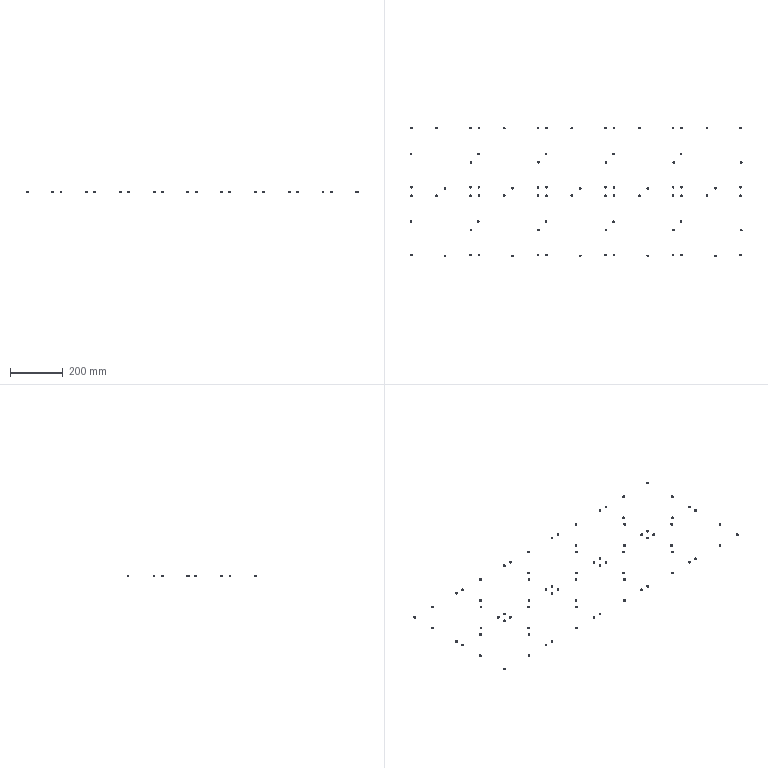Component | SolidWorks | P16BoxWeldment-1_M3RivetNut-1 | 80 solids | 480 faces | box 1258 x 490 x 3.5 mm | volume 5938 mm3 | cylinder 320 | plane 160 | commonest cylinder face diameters 3 x160 6 x160
build123d program:
from build123d import *

# Parameters (mm, degrees)
SKETCH1_R           = 3
SKETCH1_R_2         = 1.5
BOSS_EXTRUDE1_DEPTH = 3.5


with BuildPart() as part:
    # Sketch1 → Boss-Extrude1 (new body)
    # profile 1 of 80: a face of its own
    with BuildSketch(Plane.XY):
        with Locations((-352, 0)):
            Circle(SKETCH1_R)
        with Locations((-352, 0)):
            Circle(SKETCH1_R_2, mode=Mode.SUBTRACT)
    # profile 2 of 80: a face of its own
    with BuildSketch(Plane.XY):
        with Locations((-256, 0)):
            Circle(SKETCH1_R)
        with Locations((-256, 0)):
            Circle(SKETCH1_R_2, mode=Mode.SUBTRACT)
    # profile 3 of 80: a face of its own
    with BuildSketch(Plane.XY):
        with Locations((-128, 0)):
            Circle(SKETCH1_R)
        with Locations((-128, 0)):
            Circle(SKETCH1_R_2, mode=Mode.SUBTRACT)
    # profile 4 of 80: a face of its own
    with BuildSketch(Plane.XY):
        with Locations((-354, -98)):
            Circle(SKETCH1_R)
        with Locations((-354, -98)):
            Circle(SKETCH1_R_2, mode=Mode.SUBTRACT)
    # profile 5 of 80: a face of its own
    with BuildSketch(Plane.XY):
        with Locations((-126, -130)):
            Circle(SKETCH1_R)
        with Locations((-126, -130)):
            Circle(SKETCH1_R_2, mode=Mode.SUBTRACT)
    # profile 6 of 80: a face of its own
    with BuildSketch(Plane.XY):
        with Locations((-128, -224)):
            Circle(SKETCH1_R)
        with Locations((-128, -224)):
            Circle(SKETCH1_R_2, mode=Mode.SUBTRACT)
    # profile 7 of 80: a face of its own
    with BuildSketch(Plane.XY):
        with Locations((-224, -228)):
            Circle(SKETCH1_R)
        with Locations((-224, -228)):
            Circle(SKETCH1_R_2, mode=Mode.SUBTRACT)
    # profile 8 of 80: a face of its own
    with BuildSketch(Plane.XY):
        with Locations((-352, -224)):
            Circle(SKETCH1_R)
        with Locations((-352, -224)):
            Circle(SKETCH1_R_2, mode=Mode.SUBTRACT)
    # profile 9 of 80: a face of its own
    with BuildSketch(Plane.XY):
        with Locations((-96, 0)):
            Circle(SKETCH1_R)
        with Locations((-96, 0)):
            Circle(SKETCH1_R_2, mode=Mode.SUBTRACT)
    # profile 10 of 80: a face of its own
    with BuildSketch(Plane.XY):
        Circle(SKETCH1_R)
        Circle(SKETCH1_R_2, mode=Mode.SUBTRACT)
    # profile 11 of 80: a face of its own
    with BuildSketch(Plane.XY):
        with Locations((128, 0)):
            Circle(SKETCH1_R)
        with Locations((128, 0)):
            Circle(SKETCH1_R_2, mode=Mode.SUBTRACT)
    # profile 12 of 80: a face of its own
    with BuildSketch(Plane.XY):
        with Locations((-98, -98)):
            Circle(SKETCH1_R)
        with Locations((-98, -98)):
            Circle(SKETCH1_R_2, mode=Mode.SUBTRACT)
    # profile 13 of 80: a face of its own
    with BuildSketch(Plane.XY):
        with Locations((130, -130)):
            Circle(SKETCH1_R)
        with Locations((130, -130)):
            Circle(SKETCH1_R_2, mode=Mode.SUBTRACT)
    # profile 14 of 80: a face of its own
    with BuildSketch(Plane.XY):
        with Locations((128, -224)):
            Circle(SKETCH1_R)
        with Locations((128, -224)):
            Circle(SKETCH1_R_2, mode=Mode.SUBTRACT)
    # profile 15 of 80: a face of its own
    with BuildSketch(Plane.XY):
        with Locations((32, -228)):
            Circle(SKETCH1_R)
        with Locations((32, -228)):
            Circle(SKETCH1_R_2, mode=Mode.SUBTRACT)
    # profile 16 of 80: a face of its own
    with BuildSketch(Plane.XY):
        with Locations((-96, -224)):
            Circle(SKETCH1_R)
        with Locations((-96, -224)):
            Circle(SKETCH1_R_2, mode=Mode.SUBTRACT)
    # profile 17 of 80: a face of its own
    with BuildSketch(Plane.XY):
        with Locations((160, 0)):
            Circle(SKETCH1_R)
        with Locations((160, 0)):
            Circle(SKETCH1_R_2, mode=Mode.SUBTRACT)
    # profile 18 of 80: a face of its own
    with BuildSketch(Plane.XY):
        with Locations((256, 0)):
            Circle(SKETCH1_R)
        with Locations((256, 0)):
            Circle(SKETCH1_R_2, mode=Mode.SUBTRACT)
    # profile 19 of 80: a face of its own
    with BuildSketch(Plane.XY):
        with Locations((384, 0)):
            Circle(SKETCH1_R)
        with Locations((384, 0)):
            Circle(SKETCH1_R_2, mode=Mode.SUBTRACT)
    # profile 20 of 80: a face of its own
    with BuildSketch(Plane.XY):
        with Locations((158, -98)):
            Circle(SKETCH1_R)
        with Locations((158, -98)):
            Circle(SKETCH1_R_2, mode=Mode.SUBTRACT)
    # profile 21 of 80: a face of its own
    with BuildSketch(Plane.XY):
        with Locations((386, -130)):
            Circle(SKETCH1_R)
        with Locations((386, -130)):
            Circle(SKETCH1_R_2, mode=Mode.SUBTRACT)
    # profile 22 of 80: a face of its own
    with BuildSketch(Plane.XY):
        with Locations((384, -224)):
            Circle(SKETCH1_R)
        with Locations((384, -224)):
            Circle(SKETCH1_R_2, mode=Mode.SUBTRACT)
    # profile 23 of 80: a face of its own
    with BuildSketch(Plane.XY):
        with Locations((288, -228)):
            Circle(SKETCH1_R)
        with Locations((288, -228)):
            Circle(SKETCH1_R_2, mode=Mode.SUBTRACT)
    # profile 24 of 80: a face of its own
    with BuildSketch(Plane.XY):
        with Locations((160, -224)):
            Circle(SKETCH1_R)
        with Locations((160, -224)):
            Circle(SKETCH1_R_2, mode=Mode.SUBTRACT)
    # profile 25 of 80: a face of its own
    with BuildSketch(Plane.XY):
        with Locations((416, 0)):
            Circle(SKETCH1_R)
        with Locations((416, 0)):
            Circle(SKETCH1_R_2, mode=Mode.SUBTRACT)
    # profile 26 of 80: a face of its own
    with BuildSketch(Plane.XY):
        with Locations((512, 0)):
            Circle(SKETCH1_R)
        with Locations((512, 0)):
            Circle(SKETCH1_R_2, mode=Mode.SUBTRACT)
    # profile 27 of 80: a face of its own
    with BuildSketch(Plane.XY):
        with Locations((640, 0)):
            Circle(SKETCH1_R)
        with Locations((640, 0)):
            Circle(SKETCH1_R_2, mode=Mode.SUBTRACT)
    # profile 28 of 80: a face of its own
    with BuildSketch(Plane.XY):
        with Locations((414, -98)):
            Circle(SKETCH1_R)
        with Locations((414, -98)):
            Circle(SKETCH1_R_2, mode=Mode.SUBTRACT)
    # profile 29 of 80: a face of its own
    with BuildSketch(Plane.XY):
        with Locations((642, -130)):
            Circle(SKETCH1_R)
        with Locations((642, -130)):
            Circle(SKETCH1_R_2, mode=Mode.SUBTRACT)
    # profile 30 of 80: a face of its own
    with BuildSketch(Plane.XY):
        with Locations((640, -224)):
            Circle(SKETCH1_R)
        with Locations((640, -224)):
            Circle(SKETCH1_R_2, mode=Mode.SUBTRACT)
    # profile 31 of 80: a face of its own
    with BuildSketch(Plane.XY):
        with Locations((544, -228)):
            Circle(SKETCH1_R)
        with Locations((544, -228)):
            Circle(SKETCH1_R_2, mode=Mode.SUBTRACT)
    # profile 32 of 80: a face of its own
    with BuildSketch(Plane.XY):
        with Locations((416, -224)):
            Circle(SKETCH1_R)
        with Locations((416, -224)):
            Circle(SKETCH1_R_2, mode=Mode.SUBTRACT)
    # profile 33 of 80: a face of its own
    with BuildSketch(Plane.XY):
        with Locations((672, 0)):
            Circle(SKETCH1_R)
        with Locations((672, 0)):
            Circle(SKETCH1_R_2, mode=Mode.SUBTRACT)
    # profile 34 of 80: a face of its own
    with BuildSketch(Plane.XY):
        with Locations((768, 0)):
            Circle(SKETCH1_R)
        with Locations((768, 0)):
            Circle(SKETCH1_R_2, mode=Mode.SUBTRACT)
    # profile 35 of 80: a face of its own
    with BuildSketch(Plane.XY):
        with Locations((896, 0)):
            Circle(SKETCH1_R)
        with Locations((896, 0)):
            Circle(SKETCH1_R_2, mode=Mode.SUBTRACT)
    # profile 36 of 80: a face of its own
    with BuildSketch(Plane.XY):
        with Locations((670, -98)):
            Circle(SKETCH1_R)
        with Locations((670, -98)):
            Circle(SKETCH1_R_2, mode=Mode.SUBTRACT)
    # profile 37 of 80: a face of its own
    with BuildSketch(Plane.XY):
        with Locations((898, -130)):
            Circle(SKETCH1_R)
        with Locations((898, -130)):
            Circle(SKETCH1_R_2, mode=Mode.SUBTRACT)
    # profile 38 of 80: a face of its own
    with BuildSketch(Plane.XY):
        with Locations((896, -224)):
            Circle(SKETCH1_R)
        with Locations((896, -224)):
            Circle(SKETCH1_R_2, mode=Mode.SUBTRACT)
    # profile 39 of 80: a face of its own
    with BuildSketch(Plane.XY):
        with Locations((800, -228)):
            Circle(SKETCH1_R)
        with Locations((800, -228)):
            Circle(SKETCH1_R_2, mode=Mode.SUBTRACT)
    # profile 40 of 80: a face of its own
    with BuildSketch(Plane.XY):
        with Locations((672, -224)):
            Circle(SKETCH1_R)
        with Locations((672, -224)):
            Circle(SKETCH1_R_2, mode=Mode.SUBTRACT)
    # profile 41 of 80: a face of its own
    with BuildSketch(Plane.XY):
        with Locations((-352, -256)):
            Circle(SKETCH1_R)
        with Locations((-352, -256)):
            Circle(SKETCH1_R_2, mode=Mode.SUBTRACT)
    # profile 42 of 80: a face of its own
    with BuildSketch(Plane.XY):
        with Locations((-256, -256)):
            Circle(SKETCH1_R)
        with Locations((-256, -256)):
            Circle(SKETCH1_R_2, mode=Mode.SUBTRACT)
    # profile 43 of 80: a face of its own
    with BuildSketch(Plane.XY):
        with Locations((-128, -256)):
            Circle(SKETCH1_R)
        with Locations((-128, -256)):
            Circle(SKETCH1_R_2, mode=Mode.SUBTRACT)
    # profile 44 of 80: a face of its own
    with BuildSketch(Plane.XY):
        with Locations((-354, -354)):
            Circle(SKETCH1_R)
        with Locations((-354, -354)):
            Circle(SKETCH1_R_2, mode=Mode.SUBTRACT)
    # profile 45 of 80: a face of its own
    with BuildSketch(Plane.XY):
        with Locations((-126, -386)):
            Circle(SKETCH1_R)
        with Locations((-126, -386)):
            Circle(SKETCH1_R_2, mode=Mode.SUBTRACT)
    # profile 46 of 80: a face of its own
    with BuildSketch(Plane.XY):
        with Locations((-128, -480)):
            Circle(SKETCH1_R)
        with Locations((-128, -480)):
            Circle(SKETCH1_R_2, mode=Mode.SUBTRACT)
    # profile 47 of 80: a face of its own
    with BuildSketch(Plane.XY):
        with Locations((-224, -484)):
            Circle(SKETCH1_R)
        with Locations((-224, -484)):
            Circle(SKETCH1_R_2, mode=Mode.SUBTRACT)
    # profile 48 of 80: a face of its own
    with BuildSketch(Plane.XY):
        with Locations((-352, -480)):
            Circle(SKETCH1_R)
        with Locations((-352, -480)):
            Circle(SKETCH1_R_2, mode=Mode.SUBTRACT)
    # profile 49 of 80: a face of its own
    with BuildSketch(Plane.XY):
        with Locations((-96, -256)):
            Circle(SKETCH1_R)
        with Locations((-96, -256)):
            Circle(SKETCH1_R_2, mode=Mode.SUBTRACT)
    # profile 50 of 80: a face of its own
    with BuildSketch(Plane.XY):
        with Locations((0, -256)):
            Circle(SKETCH1_R)
        with Locations((0, -256)):
            Circle(SKETCH1_R_2, mode=Mode.SUBTRACT)
    # profile 51 of 80: a face of its own
    with BuildSketch(Plane.XY):
        with Locations((128, -256)):
            Circle(SKETCH1_R)
        with Locations((128, -256)):
            Circle(SKETCH1_R_2, mode=Mode.SUBTRACT)
    # profile 52 of 80: a face of its own
    with BuildSketch(Plane.XY):
        with Locations((-98, -354)):
            Circle(SKETCH1_R)
        with Locations((-98, -354)):
            Circle(SKETCH1_R_2, mode=Mode.SUBTRACT)
    # profile 53 of 80: a face of its own
    with BuildSketch(Plane.XY):
        with Locations((130, -386)):
            Circle(SKETCH1_R)
        with Locations((130, -386)):
            Circle(SKETCH1_R_2, mode=Mode.SUBTRACT)
    # profile 54 of 80: a face of its own
    with BuildSketch(Plane.XY):
        with Locations((128, -480)):
            Circle(SKETCH1_R)
        with Locations((128, -480)):
            Circle(SKETCH1_R_2, mode=Mode.SUBTRACT)
    # profile 55 of 80: a face of its own
    with BuildSketch(Plane.XY):
        with Locations((32, -484)):
            Circle(SKETCH1_R)
        with Locations((32, -484)):
            Circle(SKETCH1_R_2, mode=Mode.SUBTRACT)
    # profile 56 of 80: a face of its own
    with BuildSketch(Plane.XY):
        with Locations((-96, -480)):
            Circle(SKETCH1_R)
        with Locations((-96, -480)):
            Circle(SKETCH1_R_2, mode=Mode.SUBTRACT)
    # profile 57 of 80: a face of its own
    with BuildSketch(Plane.XY):
        with Locations((160, -256)):
            Circle(SKETCH1_R)
        with Locations((160, -256)):
            Circle(SKETCH1_R_2, mode=Mode.SUBTRACT)
    # profile 58 of 80: a face of its own
    with BuildSketch(Plane.XY):
        with Locations((256, -256)):
            Circle(SKETCH1_R)
        with Locations((256, -256)):
            Circle(SKETCH1_R_2, mode=Mode.SUBTRACT)
    # profile 59 of 80: a face of its own
    with BuildSketch(Plane.XY):
        with Locations((384, -256)):
            Circle(SKETCH1_R)
        with Locations((384, -256)):
            Circle(SKETCH1_R_2, mode=Mode.SUBTRACT)
    # profile 60 of 80: a face of its own
    with BuildSketch(Plane.XY):
        with Locations((158, -354)):
            Circle(SKETCH1_R)
        with Locations((158, -354)):
            Circle(SKETCH1_R_2, mode=Mode.SUBTRACT)
    # profile 61 of 80: a face of its own
    with BuildSketch(Plane.XY):
        with Locations((386, -386)):
            Circle(SKETCH1_R)
        with Locations((386, -386)):
            Circle(SKETCH1_R_2, mode=Mode.SUBTRACT)
    # profile 62 of 80: a face of its own
    with BuildSketch(Plane.XY):
        with Locations((384, -480)):
            Circle(SKETCH1_R)
        with Locations((384, -480)):
            Circle(SKETCH1_R_2, mode=Mode.SUBTRACT)
    # profile 63 of 80: a face of its own
    with BuildSketch(Plane.XY):
        with Locations((288, -484)):
            Circle(SKETCH1_R)
        with Locations((288, -484)):
            Circle(SKETCH1_R_2, mode=Mode.SUBTRACT)
    # profile 64 of 80: a face of its own
    with BuildSketch(Plane.XY):
        with Locations((160, -480)):
            Circle(SKETCH1_R)
        with Locations((160, -480)):
            Circle(SKETCH1_R_2, mode=Mode.SUBTRACT)
    # profile 65 of 80: a face of its own
    with BuildSketch(Plane.XY):
        with Locations((416, -256)):
            Circle(SKETCH1_R)
        with Locations((416, -256)):
            Circle(SKETCH1_R_2, mode=Mode.SUBTRACT)
    # profile 66 of 80: a face of its own
    with BuildSketch(Plane.XY):
        with Locations((512, -256)):
            Circle(SKETCH1_R)
        with Locations((512, -256)):
            Circle(SKETCH1_R_2, mode=Mode.SUBTRACT)
    # profile 67 of 80: a face of its own
    with BuildSketch(Plane.XY):
        with Locations((640, -256)):
            Circle(SKETCH1_R)
        with Locations((640, -256)):
            Circle(SKETCH1_R_2, mode=Mode.SUBTRACT)
    # profile 68 of 80: a face of its own
    with BuildSketch(Plane.XY):
        with Locations((414, -354)):
            Circle(SKETCH1_R)
        with Locations((414, -354)):
            Circle(SKETCH1_R_2, mode=Mode.SUBTRACT)
    # profile 69 of 80: a face of its own
    with BuildSketch(Plane.XY):
        with Locations((642, -386)):
            Circle(SKETCH1_R)
        with Locations((642, -386)):
            Circle(SKETCH1_R_2, mode=Mode.SUBTRACT)
    # profile 70 of 80: a face of its own
    with BuildSketch(Plane.XY):
        with Locations((640, -480)):
            Circle(SKETCH1_R)
        with Locations((640, -480)):
            Circle(SKETCH1_R_2, mode=Mode.SUBTRACT)
    # profile 71 of 80: a face of its own
    with BuildSketch(Plane.XY):
        with Locations((544, -484)):
            Circle(SKETCH1_R)
        with Locations((544, -484)):
            Circle(SKETCH1_R_2, mode=Mode.SUBTRACT)
    # profile 72 of 80: a face of its own
    with BuildSketch(Plane.XY):
        with Locations((416, -480)):
            Circle(SKETCH1_R)
        with Locations((416, -480)):
            Circle(SKETCH1_R_2, mode=Mode.SUBTRACT)
    # profile 73 of 80: a face of its own
    with BuildSketch(Plane.XY):
        with Locations((672, -256)):
            Circle(SKETCH1_R)
        with Locations((672, -256)):
            Circle(SKETCH1_R_2, mode=Mode.SUBTRACT)
    # profile 74 of 80: a face of its own
    with BuildSketch(Plane.XY):
        with Locations((768, -256)):
            Circle(SKETCH1_R)
        with Locations((768, -256)):
            Circle(SKETCH1_R_2, mode=Mode.SUBTRACT)
    # profile 75 of 80: a face of its own
    with BuildSketch(Plane.XY):
        with Locations((896, -256)):
            Circle(SKETCH1_R)
        with Locations((896, -256)):
            Circle(SKETCH1_R_2, mode=Mode.SUBTRACT)
    # profile 76 of 80: a face of its own
    with BuildSketch(Plane.XY):
        with Locations((670, -354)):
            Circle(SKETCH1_R)
        with Locations((670, -354)):
            Circle(SKETCH1_R_2, mode=Mode.SUBTRACT)
    # profile 77 of 80: a face of its own
    with BuildSketch(Plane.XY):
        with Locations((898, -386)):
            Circle(SKETCH1_R)
        with Locations((898, -386)):
            Circle(SKETCH1_R_2, mode=Mode.SUBTRACT)
    # profile 78 of 80: a face of its own
    with BuildSketch(Plane.XY):
        with Locations((896, -480)):
            Circle(SKETCH1_R)
        with Locations((896, -480)):
            Circle(SKETCH1_R_2, mode=Mode.SUBTRACT)
    # profile 79 of 80: a face of its own
    with BuildSketch(Plane.XY):
        with Locations((800, -484)):
            Circle(SKETCH1_R)
        with Locations((800, -484)):
            Circle(SKETCH1_R_2, mode=Mode.SUBTRACT)
    # profile 80 of 80: a face of its own
    with BuildSketch(Plane.XY):
        with Locations((672, -480)):
            Circle(SKETCH1_R)
        with Locations((672, -480)):
            Circle(SKETCH1_R_2, mode=Mode.SUBTRACT)
    extrude(amount=BOSS_EXTRUDE1_DEPTH)


solid = part.part

# Placed as in the assembly
solid = solid.moved(Location((-341.394, 255.542, 64.7), (0, 0, 0)))